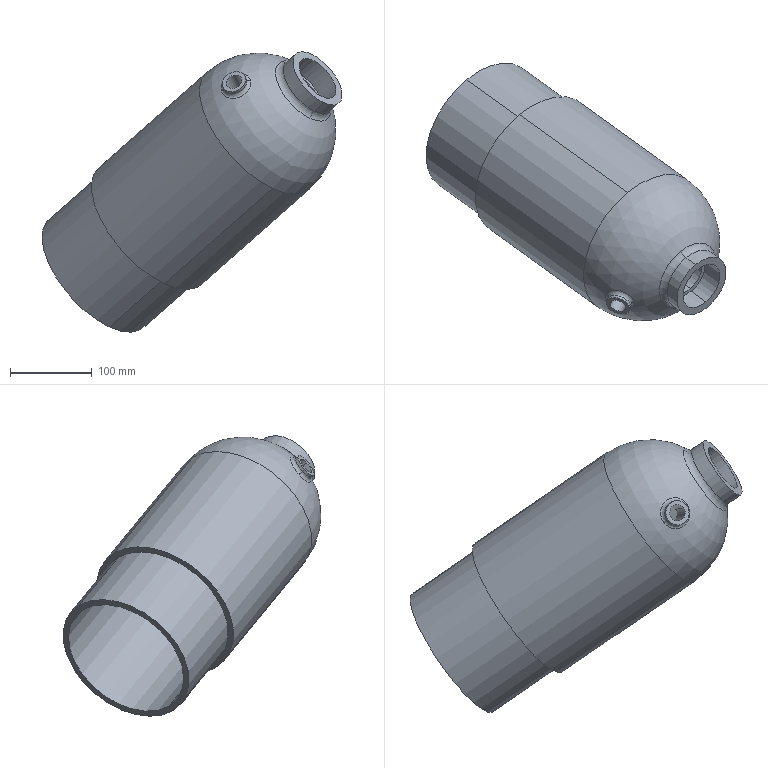Component | SolidWorks | SpringSleeve-1 | 1 solid | 35 faces | box 366.15 x 314.84 x 342.25 mm | volume 2832713 mm3 | cylinder 18 | torus 8 | plane 7 | sphere 2 | commonest cylinder face diameters 30 x4 20 x2 60 x2 175 x2 80 x2 160 x2 190 x2 50 x2 | material 201.0-T7 Insulated Mold Casting (SS)
STEP:
#1=COLOUR_RGB('',0.7922,0.8196,0.9333);
#2=FILL_AREA_STYLE_COLOUR('',#1);
#3=FILL_AREA_STYLE('',(#2));
#4=SURFACE_STYLE_FILL_AREA(#3);
#5=SURFACE_SIDE_STYLE('',(#4));
#6=SURFACE_STYLE_USAGE(.BOTH.,#5);
#7=PRESENTATION_STYLE_ASSIGNMENT((#6));
#8=CARTESIAN_POINT('',(3.904,-75.784,16.909));
#9=VERTEX_POINT('',#8);
#10=CARTESIAN_POINT('',(5.013,-75.909,17.293));
#11=VERTEX_POINT('',#10);
#12=CARTESIAN_POINT('',(4.459,-75.847,17.101));
#13=DIRECTION('',(0.2892,0.7537,-0.5902));
#14=DIRECTION('',(0.9396,-0.1055,0.3256));
#15=AXIS2_PLACEMENT_3D('',#12,#13,#14);
#16=CIRCLE('',#15,0.5906);
#17=EDGE_CURVE('',#9,#11,#16,.T.);
#18=ORIENTED_EDGE('',*,*,#17,.F.);
#19=CARTESIAN_POINT('',(3.615,-75.901,16.939));
#20=VERTEX_POINT('',#19);
#21=CARTESIAN_POINT('',(3.719,-75.764,16.844));
#22=DIRECTION('',(0.1832,-0.6488,-0.7386));
#23=DIRECTION('',(0.,0.7513,-0.6599));
#24=AXIS2_PLACEMENT_3D('',#21,#22,#23);
#25=CIRCLE('',#24,0.1969);
#26=EDGE_CURVE('',#9,#20,#25,.T.);
#27=ORIENTED_EDGE('',*,*,#26,.T.);
#28=CARTESIAN_POINT('',(5.193,-76.078,17.486));
#29=VERTEX_POINT('',#28);
#30=CARTESIAN_POINT('',(4.404,-75.99,17.213));
#31=DIRECTION('',(-0.2892,-0.7537,0.5902));
#32=DIRECTION('',(0.9396,-0.1055,0.3256));
#33=AXIS2_PLACEMENT_3D('',#30,#31,#32);
#34=CIRCLE('',#33,0.8399);
#35=EDGE_CURVE('',#29,#20,#34,.T.);
#36=ORIENTED_EDGE('',*,*,#35,.F.);
#37=CARTESIAN_POINT('',(5.198,-75.93,17.357));
#38=DIRECTION('',(-0.1832,0.6488,0.7386));
#39=DIRECTION('',(0.,-0.7513,0.6599));
#40=AXIS2_PLACEMENT_3D('',#37,#38,#39);
#41=CIRCLE('',#40,0.1969);
#42=EDGE_CURVE('',#11,#29,#41,.T.);
#43=ORIENTED_EDGE('',*,*,#42,.F.);
#44=EDGE_LOOP('',(#18,#27,#36,#43));
#45=FACE_OUTER_BOUND('',#44,.T.);
#46=CARTESIAN_POINT('',(4.459,-75.847,17.101));
#47=DIRECTION('',(0.2892,0.7537,-0.5902));
#48=DIRECTION('',(0.9396,-0.1055,0.3256));
#49=AXIS2_PLACEMENT_3D('',#46,#47,#48);
#50=TOROIDAL_SURFACE('',#49,0.7874,0.1969);
#51=ADVANCED_FACE('',(#45),#50,.F.);
#52=CARTESIAN_POINT('',(3.519,-76.385,17.341));
#53=VERTEX_POINT('',#52);
#54=CARTESIAN_POINT('',(4.925,-76.543,17.828));
#55=VERTEX_POINT('',#54);
#56=CARTESIAN_POINT('',(4.222,-76.464,17.584));
#57=DIRECTION('',(0.2892,0.7537,-0.5902));
#58=DIRECTION('',(0.9396,-0.1055,0.3256));
#59=AXIS2_PLACEMENT_3D('',#56,#57,#58);
#60=CIRCLE('',#59,0.748);
#61=EDGE_CURVE('',#53,#55,#60,.T.);
#62=ORIENTED_EDGE('',*,*,#61,.F.);
#63=CARTESIAN_POINT('',(3.611,-76.547,17.506));
#64=VERTEX_POINT('',#63);
#65=CARTESIAN_POINT('',(3.426,-76.526,17.442));
#66=DIRECTION('',(0.1832,-0.6488,-0.7386));
#67=DIRECTION('',(0.,0.7513,-0.6599));
#68=AXIS2_PLACEMENT_3D('',#65,#66,#67);
#69=CIRCLE('',#68,0.1969);
#70=EDGE_CURVE('',#53,#64,#69,.T.);
#71=ORIENTED_EDGE('',*,*,#70,.T.);
#72=CARTESIAN_POINT('',(4.721,-76.671,17.89));
#73=VERTEX_POINT('',#72);
#74=CARTESIAN_POINT('',(4.166,-76.609,17.698));
#75=DIRECTION('',(-0.2892,-0.7537,0.5902));
#76=DIRECTION('',(0.9396,-0.1055,0.3256));
#77=AXIS2_PLACEMENT_3D('',#74,#75,#76);
#78=CIRCLE('',#77,0.5906);
#79=EDGE_CURVE('',#73,#64,#78,.T.);
#80=ORIENTED_EDGE('',*,*,#79,.F.);
#81=CARTESIAN_POINT('',(4.906,-76.692,17.954));
#82=DIRECTION('',(-0.1832,0.6488,0.7386));
#83=DIRECTION('',(0.,-0.7513,0.6599));
#84=AXIS2_PLACEMENT_3D('',#81,#82,#83);
#85=CIRCLE('',#84,0.1969);
#86=EDGE_CURVE('',#55,#73,#85,.T.);
#87=ORIENTED_EDGE('',*,*,#86,.F.);
#88=EDGE_LOOP('',(#62,#71,#80,#87));
#89=FACE_OUTER_BOUND('',#88,.T.);
#90=CARTESIAN_POINT('',(4.166,-76.609,17.698));
#91=DIRECTION('',(0.2892,0.7537,-0.5902));
#92=DIRECTION('',(0.9396,-0.1055,0.3256));
#93=AXIS2_PLACEMENT_3D('',#90,#91,#92);
#94=TOROIDAL_SURFACE('',#93,0.7874,0.1969);
#95=ADVANCED_FACE('',(#89),#94,.F.);
#96=CARTESIAN_POINT('',(4.096,-75.785,16.957));
#97=VERTEX_POINT('',#96);
#98=CARTESIAN_POINT('',(4.836,-75.868,17.214));
#99=VERTEX_POINT('',#98);
#100=CARTESIAN_POINT('',(4.466,-75.827,17.085));
#101=DIRECTION('',(0.2892,0.7537,-0.5902));
#102=DIRECTION('',(0.9396,-0.1055,0.3256));
#103=AXIS2_PLACEMENT_3D('',#100,#101,#102);
#104=CIRCLE('',#103,0.3937);
#105=EDGE_CURVE('',#97,#99,#104,.T.);
#106=ORIENTED_EDGE('',*,*,#105,.T.);
#107=CARTESIAN_POINT('',(4.494,-76.759,17.911));
#108=VERTEX_POINT('',#107);
#109=CARTESIAN_POINT('',(4.836,-75.868,17.214));
#110=DIRECTION('',(-0.2892,-0.7537,0.5902));
#111=VECTOR('',#110,39.37);
#112=LINE('',#109,#111);
#113=EDGE_CURVE('',#99,#108,#112,.T.);
#114=ORIENTED_EDGE('',*,*,#113,.T.);
#115=CARTESIAN_POINT('',(3.755,-76.675,17.654));
#116=VERTEX_POINT('',#115);
#117=CARTESIAN_POINT('',(4.125,-76.717,17.782));
#118=DIRECTION('',(0.2892,0.7537,-0.5902));
#119=DIRECTION('',(0.9396,-0.1055,0.3256));
#120=AXIS2_PLACEMENT_3D('',#117,#118,#119);
#121=CIRCLE('',#120,0.3937);
#122=EDGE_CURVE('',#116,#108,#121,.T.);
#123=ORIENTED_EDGE('',*,*,#122,.F.);
#124=CARTESIAN_POINT('',(4.096,-75.785,16.957));
#125=DIRECTION('',(-0.2892,-0.7537,0.5902));
#126=VECTOR('',#125,39.37);
#127=LINE('',#124,#126);
#128=EDGE_CURVE('',#97,#116,#127,.T.);
#129=ORIENTED_EDGE('',*,*,#128,.F.);
#130=EDGE_LOOP('',(#106,#114,#123,#129));
#131=FACE_OUTER_BOUND('',#130,.T.);
#132=CARTESIAN_POINT('',(4.466,-75.827,17.085));
#133=DIRECTION('',(-0.2892,-0.7537,0.5902));
#134=DIRECTION('',(-0.9396,0.1055,-0.3256));
#135=AXIS2_PLACEMENT_3D('',#132,#133,#134);
#136=CYLINDRICAL_SURFACE('',#135,0.3937);
#137=ADVANCED_FACE('',(#131),#136,.F.);
#138=CARTESIAN_POINT('',(4.459,-75.847,17.101));
#139=DIRECTION('',(0.2892,0.7537,-0.5902));
#140=DIRECTION('',(0.9396,-0.1055,0.3256));
#141=AXIS2_PLACEMENT_3D('',#138,#139,#140);
#142=CIRCLE('',#141,0.5906);
#143=EDGE_CURVE('',#11,#9,#142,.T.);
#144=ORIENTED_EDGE('',*,*,#143,.T.);
#145=CARTESIAN_POINT('',(3.911,-75.765,16.893));
#146=VERTEX_POINT('',#145);
#147=CARTESIAN_POINT('',(3.57,-76.655,17.59));
#148=DIRECTION('',(0.2892,0.7537,-0.5902));
#149=VECTOR('',#148,39.37);
#150=LINE('',#147,#149);
#151=EDGE_CURVE('',#9,#146,#150,.T.);
#152=ORIENTED_EDGE('',*,*,#151,.T.);
#153=CARTESIAN_POINT('',(5.021,-75.889,17.278));
#154=VERTEX_POINT('',#153);
#155=CARTESIAN_POINT('',(4.466,-75.827,17.085));
#156=DIRECTION('',(0.2892,0.7537,-0.5902));
#157=DIRECTION('',(0.9396,-0.1055,0.3256));
#158=AXIS2_PLACEMENT_3D('',#155,#156,#157);
#159=CIRCLE('',#158,0.5906);
#160=EDGE_CURVE('',#154,#146,#159,.T.);
#161=ORIENTED_EDGE('',*,*,#160,.F.);
#162=CARTESIAN_POINT('',(4.679,-76.779,17.975));
#163=DIRECTION('',(0.2892,0.7537,-0.5902));
#164=VECTOR('',#163,39.37);
#165=LINE('',#162,#164);
#166=EDGE_CURVE('',#11,#154,#165,.T.);
#167=ORIENTED_EDGE('',*,*,#166,.F.);
#168=EDGE_LOOP('',(#144,#152,#161,#167));
#169=FACE_OUTER_BOUND('',#168,.T.);
#170=CARTESIAN_POINT('',(4.125,-76.717,17.782));
#171=DIRECTION('',(0.2892,0.7537,-0.5902));
#172=DIRECTION('',(0.9396,-0.1055,0.3256));
#173=AXIS2_PLACEMENT_3D('',#170,#171,#172);
#174=CYLINDRICAL_SURFACE('',#173,0.5906);
#175=ADVANCED_FACE('',(#169),#174,.T.);
#176=CARTESIAN_POINT('',(4.679,-76.779,17.975));
#177=VERTEX_POINT('',#176);
#178=CARTESIAN_POINT('',(3.57,-76.655,17.59));
#179=VERTEX_POINT('',#178);
#180=CARTESIAN_POINT('',(4.125,-76.717,17.782));
#181=DIRECTION('',(0.2892,0.7537,-0.5902));
#182=DIRECTION('',(0.9396,-0.1055,0.3256));
#183=AXIS2_PLACEMENT_3D('',#180,#181,#182);
#184=CIRCLE('',#183,0.5906);
#185=EDGE_CURVE('',#177,#179,#184,.T.);
#186=ORIENTED_EDGE('',*,*,#185,.T.);
#187=CARTESIAN_POINT('',(3.57,-76.655,17.59));
#188=DIRECTION('',(0.2892,0.7537,-0.5902));
#189=VECTOR('',#188,39.37);
#190=LINE('',#187,#189);
#191=EDGE_CURVE('',#179,#64,#190,.T.);
#192=ORIENTED_EDGE('',*,*,#191,.T.);
#193=CARTESIAN_POINT('',(4.166,-76.609,17.698));
#194=DIRECTION('',(-0.2892,-0.7537,0.5902));
#195=DIRECTION('',(0.9396,-0.1055,0.3256));
#196=AXIS2_PLACEMENT_3D('',#193,#194,#195);
#197=CIRCLE('',#196,0.5906);
#198=EDGE_CURVE('',#64,#73,#197,.T.);
#199=ORIENTED_EDGE('',*,*,#198,.T.);
#200=CARTESIAN_POINT('',(4.679,-76.779,17.975));
#201=DIRECTION('',(0.2892,0.7537,-0.5902));
#202=VECTOR('',#201,39.37);
#203=LINE('',#200,#202);
#204=EDGE_CURVE('',#177,#73,#203,.T.);
#205=ORIENTED_EDGE('',*,*,#204,.F.);
#206=EDGE_LOOP('',(#186,#192,#199,#205));
#207=FACE_OUTER_BOUND('',#206,.T.);
#208=CARTESIAN_POINT('',(4.125,-76.717,17.782));
#209=DIRECTION('',(0.2892,0.7537,-0.5902));
#210=DIRECTION('',(0.9396,-0.1055,0.3256));
#211=AXIS2_PLACEMENT_3D('',#208,#209,#210);
#212=CYLINDRICAL_SURFACE('',#211,0.5906);
#213=ADVANCED_FACE('',(#207),#212,.T.);
#214=CARTESIAN_POINT('',(7.639,-76.015,16.439));
#215=VERTEX_POINT('',#214);
#216=CARTESIAN_POINT('',(7.206,-74.483,18.183));
#217=VERTEX_POINT('',#216);
#218=CARTESIAN_POINT('',(7.423,-75.249,17.311));
#219=DIRECTION('',(0.6592,-0.4763,0.5818));
#220=DIRECTION('',(-0.1832,0.6488,0.7386));
#221=AXIS2_PLACEMENT_3D('',#218,#219,#220);
#222=CIRCLE('',#221,1.181);
#223=EDGE_CURVE('',#215,#217,#222,.T.);
#224=ORIENTED_EDGE('',*,*,#223,.F.);
#225=CARTESIAN_POINT('',(8.353,-76.531,17.069));
#226=VERTEX_POINT('',#225);
#227=CARTESIAN_POINT('',(7.639,-76.015,16.439));
#228=DIRECTION('',(0.6592,-0.4763,0.5818));
#229=VECTOR('',#228,39.37);
#230=LINE('',#227,#229);
#231=EDGE_CURVE('',#215,#226,#230,.T.);
#232=ORIENTED_EDGE('',*,*,#231,.T.);
#233=CARTESIAN_POINT('',(7.92,-74.999,18.813));
#234=VERTEX_POINT('',#233);
#235=CARTESIAN_POINT('',(8.136,-75.765,17.941));
#236=DIRECTION('',(0.6592,-0.4763,0.5818));
#237=DIRECTION('',(-0.1832,0.6488,0.7386));
#238=AXIS2_PLACEMENT_3D('',#235,#236,#237);
#239=CIRCLE('',#238,1.181);
#240=EDGE_CURVE('',#226,#234,#239,.T.);
#241=ORIENTED_EDGE('',*,*,#240,.T.);
#242=CARTESIAN_POINT('',(7.206,-74.483,18.183));
#243=DIRECTION('',(0.6592,-0.4763,0.5818));
#244=VECTOR('',#243,39.37);
#245=LINE('',#242,#244);
#246=EDGE_CURVE('',#217,#234,#245,.T.);
#247=ORIENTED_EDGE('',*,*,#246,.F.);
#248=EDGE_LOOP('',(#224,#232,#241,#247));
#249=FACE_OUTER_BOUND('',#248,.T.);
#250=CARTESIAN_POINT('',(7.423,-75.249,17.311));
#251=DIRECTION('',(0.6592,-0.4763,0.5818));
#252=DIRECTION('',(-0.1832,0.6488,0.7386));
#253=AXIS2_PLACEMENT_3D('',#250,#251,#252);
#254=CYLINDRICAL_SURFACE('',#253,1.181);
#255=ADVANCED_FACE('',(#249),#254,.F.);
#256=CARTESIAN_POINT('',(7.123,-74.113,18.65));
#257=VERTEX_POINT('',#256);
#258=CARTESIAN_POINT('',(7.776,-76.424,16.019));
#259=VERTEX_POINT('',#258);
#260=CARTESIAN_POINT('',(7.45,-75.269,17.335));
#261=DIRECTION('',(-0.6592,0.4763,-0.5818));
#262=DIRECTION('',(0.1832,-0.6488,-0.7386));
#263=AXIS2_PLACEMENT_3D('',#260,#261,#262);
#264=CIRCLE('',#263,1.781);
#265=EDGE_CURVE('',#257,#259,#264,.T.);
#266=ORIENTED_EDGE('',*,*,#265,.F.);
#267=CARTESIAN_POINT('',(7.389,-74.412,18.699));
#268=VERTEX_POINT('',#267);
#269=CARTESIAN_POINT('',(7.317,-74.156,18.99));
#270=DIRECTION('',(-0.7293,-0.5935,0.3404));
#271=DIRECTION('',(0.6312,-0.7756,0.));
#272=AXIS2_PLACEMENT_3D('',#269,#270,#271);
#273=CIRCLE('',#272,0.3937);
#274=EDGE_CURVE('',#257,#268,#273,.T.);
#275=ORIENTED_EDGE('',*,*,#274,.T.);
#276=CARTESIAN_POINT('',(7.966,-76.455,16.373));
#277=VERTEX_POINT('',#276);
#278=CARTESIAN_POINT('',(7.678,-75.433,17.536));
#279=DIRECTION('',(0.6592,-0.4763,0.5818));
#280=DIRECTION('',(0.1832,-0.6488,-0.7386));
#281=AXIS2_PLACEMENT_3D('',#278,#279,#280);
#282=CIRCLE('',#281,1.575);
#283=EDGE_CURVE('',#277,#268,#282,.T.);
#284=ORIENTED_EDGE('',*,*,#283,.F.);
#285=CARTESIAN_POINT('',(8.038,-76.71,16.082));
#286=DIRECTION('',(0.7293,0.5935,-0.3404));
#287=DIRECTION('',(-0.6312,0.7756,0.));
#288=AXIS2_PLACEMENT_3D('',#285,#286,#287);
#289=CIRCLE('',#288,0.3937);
#290=EDGE_CURVE('',#259,#277,#289,.T.);
#291=ORIENTED_EDGE('',*,*,#290,.F.);
#292=EDGE_LOOP('',(#266,#275,#284,#291));
#293=FACE_OUTER_BOUND('',#292,.T.);
#294=CARTESIAN_POINT('',(7.678,-75.433,17.536));
#295=DIRECTION('',(-0.6592,0.4763,-0.5818));
#296=DIRECTION('',(0.1832,-0.6488,-0.7386));
#297=AXIS2_PLACEMENT_3D('',#294,#295,#296);
#298=TOROIDAL_SURFACE('',#297,1.969,0.3937);
#299=ADVANCED_FACE('',(#293),#298,.F.);
#300=CARTESIAN_POINT('',(6.55,-73.805,17.959));
#301=VERTEX_POINT('',#300);
#302=CARTESIAN_POINT('',(7.127,-75.849,15.632));
#303=VERTEX_POINT('',#302);
#304=CARTESIAN_POINT('',(6.839,-74.827,16.796));
#305=DIRECTION('',(-0.6592,0.4763,-0.5818));
#306=DIRECTION('',(0.1832,-0.6488,-0.7386));
#307=AXIS2_PLACEMENT_3D('',#304,#305,#306);
#308=CIRCLE('',#307,1.575);
#309=EDGE_CURVE('',#301,#303,#308,.T.);
#310=ORIENTED_EDGE('',*,*,#309,.F.);
#311=CARTESIAN_POINT('',(6.452,-73.468,18.336));
#312=VERTEX_POINT('',#311);
#313=CARTESIAN_POINT('',(6.306,-73.497,17.972));
#314=DIRECTION('',(-0.7293,-0.5935,0.3404));
#315=DIRECTION('',(0.6312,-0.7756,0.));
#316=AXIS2_PLACEMENT_3D('',#313,#314,#315);
#317=CIRCLE('',#316,0.3937);
#318=EDGE_CURVE('',#301,#312,#317,.T.);
#319=ORIENTED_EDGE('',*,*,#318,.T.);
#320=CARTESIAN_POINT('',(7.218,-76.18,15.248));
#321=VERTEX_POINT('',#320);
#322=CARTESIAN_POINT('',(6.835,-74.824,16.792));
#323=DIRECTION('',(0.6592,-0.4763,0.5818));
#324=DIRECTION('',(0.1832,-0.6488,-0.7386));
#325=AXIS2_PLACEMENT_3D('',#322,#323,#324);
#326=CIRCLE('',#325,2.09);
#327=EDGE_CURVE('',#321,#312,#326,.T.);
#328=ORIENTED_EDGE('',*,*,#327,.F.);
#329=CARTESIAN_POINT('',(6.976,-75.87,15.27));
#330=DIRECTION('',(0.7293,0.5935,-0.3404));
#331=DIRECTION('',(-0.6312,0.7756,0.));
#332=AXIS2_PLACEMENT_3D('',#329,#330,#331);
#333=CIRCLE('',#332,0.3937);
#334=EDGE_CURVE('',#303,#321,#333,.T.);
#335=ORIENTED_EDGE('',*,*,#334,.F.);
#336=EDGE_LOOP('',(#310,#319,#328,#335));
#337=FACE_OUTER_BOUND('',#336,.T.);
#338=CARTESIAN_POINT('',(6.641,-74.684,16.621));
#339=DIRECTION('',(-0.6592,0.4763,-0.5818));
#340=DIRECTION('',(0.1832,-0.6488,-0.7386));
#341=AXIS2_PLACEMENT_3D('',#338,#339,#340);
#342=TOROIDAL_SURFACE('',#341,1.829,0.3937);
#343=ADVANCED_FACE('',(#337),#342,.F.);
#344=CARTESIAN_POINT('',(-1.874,-70.311,6.005));
#345=VERTEX_POINT('',#344);
#346=CARTESIAN_POINT('',(-3.135,-65.841,11.094));
#347=VERTEX_POINT('',#346);
#348=CARTESIAN_POINT('',(-2.505,-68.076,8.549));
#349=DIRECTION('',(-0.6592,0.4763,-0.5818));
#350=DIRECTION('',(0.1832,-0.6488,-0.7386));
#351=AXIS2_PLACEMENT_3D('',#348,#349,#350);
#352=CIRCLE('',#351,3.445);
#353=EDGE_CURVE('',#345,#347,#352,.T.);
#354=ORIENTED_EDGE('',*,*,#353,.F.);
#355=CARTESIAN_POINT('',(0.7217,-72.186,8.295));
#356=VERTEX_POINT('',#355);
#357=CARTESIAN_POINT('',(-1.874,-70.311,6.005));
#358=DIRECTION('',(0.6592,-0.4763,0.5818));
#359=VECTOR('',#358,39.37);
#360=LINE('',#357,#359);
#361=EDGE_CURVE('',#345,#356,#360,.T.);
#362=ORIENTED_EDGE('',*,*,#361,.T.);
#363=CARTESIAN_POINT('',(-0.5401,-67.716,13.384));
#364=VERTEX_POINT('',#363);
#365=CARTESIAN_POINT('',(0.09081,-69.951,10.84));
#366=DIRECTION('',(-0.6592,0.4763,-0.5818));
#367=DIRECTION('',(0.1832,-0.6488,-0.7386));
#368=AXIS2_PLACEMENT_3D('',#365,#366,#367);
#369=CIRCLE('',#368,3.445);
#370=EDGE_CURVE('',#356,#364,#369,.T.);
#371=ORIENTED_EDGE('',*,*,#370,.T.);
#372=CARTESIAN_POINT('',(-3.135,-65.841,11.094));
#373=DIRECTION('',(0.6592,-0.4763,0.5818));
#374=VECTOR('',#373,39.37);
#375=LINE('',#372,#374);
#376=EDGE_CURVE('',#347,#364,#375,.T.);
#377=ORIENTED_EDGE('',*,*,#376,.F.);
#378=EDGE_LOOP('',(#354,#362,#371,#377));
#379=FACE_OUTER_BOUND('',#378,.T.);
#380=CARTESIAN_POINT('',(-2.505,-68.076,8.549));
#381=DIRECTION('',(0.6592,-0.4763,0.5818));
#382=DIRECTION('',(-0.1832,0.6488,0.7386));
#383=AXIS2_PLACEMENT_3D('',#380,#381,#382);
#384=CYLINDRICAL_SURFACE('',#383,3.445);
#385=ADVANCED_FACE('',(#379),#384,.T.);
#386=CARTESIAN_POINT('',(7.678,-75.433,17.536));
#387=DIRECTION('',(0.6592,-0.4763,0.5818));
#388=DIRECTION('',(0.1832,-0.6488,-0.7386));
#389=AXIS2_PLACEMENT_3D('',#386,#387,#388);
#390=CIRCLE('',#389,1.575);
#391=EDGE_CURVE('',#268,#277,#390,.T.);
#392=ORIENTED_EDGE('',*,*,#391,.T.);
#393=CARTESIAN_POINT('',(8.425,-76.786,16.778));
#394=VERTEX_POINT('',#393);
#395=CARTESIAN_POINT('',(7.127,-75.849,15.632));
#396=DIRECTION('',(0.6592,-0.4763,0.5818));
#397=VECTOR('',#396,39.37);
#398=LINE('',#395,#397);
#399=EDGE_CURVE('',#277,#394,#398,.T.);
#400=ORIENTED_EDGE('',*,*,#399,.T.);
#401=CARTESIAN_POINT('',(7.848,-74.743,19.104));
#402=VERTEX_POINT('',#401);
#403=CARTESIAN_POINT('',(8.136,-75.765,17.941));
#404=DIRECTION('',(-0.6592,0.4763,-0.5818));
#405=DIRECTION('',(0.1832,-0.6488,-0.7386));
#406=AXIS2_PLACEMENT_3D('',#403,#404,#405);
#407=CIRCLE('',#406,1.575);
#408=EDGE_CURVE('',#394,#402,#407,.T.);
#409=ORIENTED_EDGE('',*,*,#408,.T.);
#410=CARTESIAN_POINT('',(6.55,-73.805,17.959));
#411=DIRECTION('',(0.6592,-0.4763,0.5818));
#412=VECTOR('',#411,39.37);
#413=LINE('',#410,#412);
#414=EDGE_CURVE('',#268,#402,#413,.T.);
#415=ORIENTED_EDGE('',*,*,#414,.F.);
#416=EDGE_LOOP('',(#392,#400,#409,#415));
#417=FACE_OUTER_BOUND('',#416,.T.);
#418=CARTESIAN_POINT('',(6.839,-74.827,16.796));
#419=DIRECTION('',(0.6592,-0.4763,0.5818));
#420=DIRECTION('',(-0.1832,0.6488,0.7386));
#421=AXIS2_PLACEMENT_3D('',#418,#419,#420);
#422=CYLINDRICAL_SURFACE('',#421,1.575);
#423=ADVANCED_FACE('',(#417),#422,.T.);
#424=CARTESIAN_POINT('',(-3.081,-66.033,10.875));
#425=VERTEX_POINT('',#424);
#426=CARTESIAN_POINT('',(-1.928,-70.119,6.223));
#427=VERTEX_POINT('',#426);
#428=CARTESIAN_POINT('',(-2.505,-68.076,8.549));
#429=DIRECTION('',(-0.6592,0.4763,-0.5818));
#430=DIRECTION('',(0.1832,-0.6488,-0.7386));
#431=AXIS2_PLACEMENT_3D('',#428,#429,#430);
#432=CIRCLE('',#431,3.15);
#433=EDGE_CURVE('',#425,#427,#432,.T.);
#434=ORIENTED_EDGE('',*,*,#433,.T.);
#435=CARTESIAN_POINT('',(5.858,-75.745,13.095));
#436=VERTEX_POINT('',#435);
#437=CARTESIAN_POINT('',(-1.928,-70.119,6.223));
#438=DIRECTION('',(0.6592,-0.4763,0.5818));
#439=VECTOR('',#438,39.37);
#440=LINE('',#437,#439);
#441=EDGE_CURVE('',#427,#436,#440,.T.);
#442=ORIENTED_EDGE('',*,*,#441,.T.);
#443=CARTESIAN_POINT('',(4.705,-71.659,17.748));
#444=VERTEX_POINT('',#443);
#445=CARTESIAN_POINT('',(5.282,-73.702,15.421));
#446=DIRECTION('',(-0.6592,0.4763,-0.5818));
#447=DIRECTION('',(0.1832,-0.6488,-0.7386));
#448=AXIS2_PLACEMENT_3D('',#445,#446,#447);
#449=CIRCLE('',#448,3.15);
#450=EDGE_CURVE('',#444,#436,#449,.T.);
#451=ORIENTED_EDGE('',*,*,#450,.F.);
#452=CARTESIAN_POINT('',(-3.081,-66.033,10.875));
#453=DIRECTION('',(0.6592,-0.4763,0.5818));
#454=VECTOR('',#453,39.37);
#455=LINE('',#452,#454);
#456=EDGE_CURVE('',#425,#444,#455,.T.);
#457=ORIENTED_EDGE('',*,*,#456,.F.);
#458=EDGE_LOOP('',(#434,#442,#451,#457));
#459=FACE_OUTER_BOUND('',#458,.T.);
#460=CARTESIAN_POINT('',(-2.505,-68.076,8.549));
#461=DIRECTION('',(0.6592,-0.4763,0.5818));
#462=DIRECTION('',(-0.1832,0.6488,0.7386));
#463=AXIS2_PLACEMENT_3D('',#460,#461,#462);
#464=CYLINDRICAL_SURFACE('',#463,3.15);
#465=ADVANCED_FACE('',(#459),#464,.F.);
#466=CARTESIAN_POINT('',(0.7758,-72.378,8.077));
#467=VERTEX_POINT('',#466);
#468=CARTESIAN_POINT('',(-0.5942,-67.525,13.602));
#469=VERTEX_POINT('',#468);
#470=CARTESIAN_POINT('',(0.09081,-69.951,10.84));
#471=DIRECTION('',(-0.6592,0.4763,-0.5818));
#472=DIRECTION('',(0.1832,-0.6488,-0.7386));
#473=AXIS2_PLACEMENT_3D('',#470,#471,#472);
#474=CIRCLE('',#473,3.74);
#475=EDGE_CURVE('',#467,#469,#474,.T.);
#476=ORIENTED_EDGE('',*,*,#475,.F.);
#477=CARTESIAN_POINT('',(5.967,-76.128,12.659));
#478=VERTEX_POINT('',#477);
#479=CARTESIAN_POINT('',(-1.82,-70.502,5.786));
#480=DIRECTION('',(0.6592,-0.4763,0.5818));
#481=VECTOR('',#480,39.37);
#482=LINE('',#479,#481);
#483=EDGE_CURVE('',#467,#478,#482,.T.);
#484=ORIENTED_EDGE('',*,*,#483,.T.);
#485=CARTESIAN_POINT('',(4.597,-71.275,18.184));
#486=VERTEX_POINT('',#485);
#487=CARTESIAN_POINT('',(5.282,-73.702,15.421));
#488=DIRECTION('',(-0.6592,0.4763,-0.5818));
#489=DIRECTION('',(0.7293,0.5935,-0.3404));
#490=AXIS2_PLACEMENT_3D('',#487,#488,#489);
#491=CIRCLE('',#490,3.74);
#492=EDGE_CURVE('',#478,#486,#491,.T.);
#493=ORIENTED_EDGE('',*,*,#492,.T.);
#494=CARTESIAN_POINT('',(-3.19,-65.649,11.312));
#495=DIRECTION('',(0.6592,-0.4763,0.5818));
#496=VECTOR('',#495,39.37);
#497=LINE('',#494,#496);
#498=EDGE_CURVE('',#469,#486,#497,.T.);
#499=ORIENTED_EDGE('',*,*,#498,.F.);
#500=EDGE_LOOP('',(#476,#484,#493,#499));
#501=FACE_OUTER_BOUND('',#500,.T.);
#502=CARTESIAN_POINT('',(-2.505,-68.076,8.549));
#503=DIRECTION('',(0.6592,-0.4763,0.5818));
#504=DIRECTION('',(-0.1832,0.6488,0.7386));
#505=AXIS2_PLACEMENT_3D('',#502,#503,#504);
#506=CYLINDRICAL_SURFACE('',#505,3.74);
#507=ADVANCED_FACE('',(#501),#506,.T.);
#508=CARTESIAN_POINT('',(6.658,-74.189,17.523));
#509=VERTEX_POINT('',#508);
#510=CARTESIAN_POINT('',(7.019,-75.466,16.069));
#511=VERTEX_POINT('',#510);
#512=CARTESIAN_POINT('',(6.839,-74.827,16.796));
#513=DIRECTION('',(-0.6592,0.4763,-0.5818));
#514=DIRECTION('',(0.1832,-0.6488,-0.7386));
#515=AXIS2_PLACEMENT_3D('',#512,#513,#514);
#516=CIRCLE('',#515,0.9843);
#517=EDGE_CURVE('',#509,#511,#516,.T.);
#518=ORIENTED_EDGE('',*,*,#517,.T.);
#519=CARTESIAN_POINT('',(7.603,-75.888,16.584));
#520=VERTEX_POINT('',#519);
#521=CARTESIAN_POINT('',(6.63,-75.184,15.725));
#522=DIRECTION('',(0.6592,-0.4763,0.5818));
#523=VECTOR('',#522,39.37);
#524=LINE('',#521,#523);
#525=EDGE_CURVE('',#511,#520,#524,.T.);
#526=ORIENTED_EDGE('',*,*,#525,.T.);
#527=CARTESIAN_POINT('',(7.242,-74.611,18.038));
#528=VERTEX_POINT('',#527);
#529=CARTESIAN_POINT('',(7.423,-75.249,17.311));
#530=DIRECTION('',(-0.6592,0.4763,-0.5818));
#531=DIRECTION('',(-0.1832,0.6488,0.7386));
#532=AXIS2_PLACEMENT_3D('',#529,#530,#531);
#533=CIRCLE('',#532,0.9843);
#534=EDGE_CURVE('',#528,#520,#533,.T.);
#535=ORIENTED_EDGE('',*,*,#534,.F.);
#536=CARTESIAN_POINT('',(6.269,-73.907,17.179));
#537=DIRECTION('',(0.6592,-0.4763,0.5818));
#538=VECTOR('',#537,39.37);
#539=LINE('',#536,#538);
#540=EDGE_CURVE('',#509,#528,#539,.T.);
#541=ORIENTED_EDGE('',*,*,#540,.F.);
#542=EDGE_LOOP('',(#518,#526,#535,#541));
#543=FACE_OUTER_BOUND('',#542,.T.);
#544=CARTESIAN_POINT('',(6.449,-74.546,16.452));
#545=DIRECTION('',(0.6592,-0.4763,0.5818));
#546=DIRECTION('',(-0.1832,0.6488,0.7386));
#547=AXIS2_PLACEMENT_3D('',#544,#545,#546);
#548=CYLINDRICAL_SURFACE('',#547,0.9843);
#549=ADVANCED_FACE('',(#543),#548,.F.);
#550=ORIENTED_EDGE('',*,*,#525,.F.);
#551=CARTESIAN_POINT('',(6.839,-74.827,16.796));
#552=DIRECTION('',(-0.6592,0.4763,-0.5818));
#553=DIRECTION('',(0.1832,-0.6488,-0.7386));
#554=AXIS2_PLACEMENT_3D('',#551,#552,#553);
#555=CIRCLE('',#554,0.9843);
#556=EDGE_CURVE('',#511,#509,#555,.T.);
#557=ORIENTED_EDGE('',*,*,#556,.T.);
#558=ORIENTED_EDGE('',*,*,#540,.T.);
#559=CARTESIAN_POINT('',(7.423,-75.249,17.311));
#560=DIRECTION('',(-0.6592,0.4763,-0.5818));
#561=DIRECTION('',(-0.1832,0.6488,0.7386));
#562=AXIS2_PLACEMENT_3D('',#559,#560,#561);
#563=CIRCLE('',#562,0.9843);
#564=EDGE_CURVE('',#520,#528,#563,.T.);
#565=ORIENTED_EDGE('',*,*,#564,.F.);
#566=EDGE_LOOP('',(#550,#557,#558,#565));
#567=FACE_OUTER_BOUND('',#566,.T.);
#568=CARTESIAN_POINT('',(6.449,-74.546,16.452));
#569=DIRECTION('',(0.6592,-0.4763,0.5818));
#570=DIRECTION('',(-0.1832,0.6488,0.7386));
#571=AXIS2_PLACEMENT_3D('',#568,#569,#570);
#572=CYLINDRICAL_SURFACE('',#571,0.9843);
#573=ADVANCED_FACE('',(#567),#572,.F.);
#574=ORIENTED_EDGE('',*,*,#433,.F.);
#575=CARTESIAN_POINT('',(-2.505,-68.076,8.549));
#576=DIRECTION('',(-0.6592,0.4763,-0.5818));
#577=DIRECTION('',(0.1832,-0.6488,-0.7386));
#578=AXIS2_PLACEMENT_3D('',#575,#576,#577);
#579=CIRCLE('',#578,3.15);
#580=EDGE_CURVE('',#427,#425,#579,.T.);
#581=ORIENTED_EDGE('',*,*,#580,.F.);
#582=EDGE_LOOP('',(#574,#581));
#583=FACE_BOUND('',#582,.T.);
#584=CARTESIAN_POINT('',(-2.505,-68.076,8.549));
#585=DIRECTION('',(-0.6592,0.4763,-0.5818));
#586=DIRECTION('',(0.1832,-0.6488,-0.7386));
#587=AXIS2_PLACEMENT_3D('',#584,#585,#586);
#588=CIRCLE('',#587,3.445);
#589=EDGE_CURVE('',#347,#345,#588,.T.);
#590=ORIENTED_EDGE('',*,*,#589,.T.);
#591=ORIENTED_EDGE('',*,*,#353,.T.);
#592=EDGE_LOOP('',(#590,#591));
#593=FACE_OUTER_BOUND('',#592,.T.);
#594=CARTESIAN_POINT('',(-2.505,-68.076,8.549));
#595=DIRECTION('',(-0.6592,0.4763,-0.5818));
#596=DIRECTION('',(0.1832,-0.6488,-0.7386));
#597=AXIS2_PLACEMENT_3D('',#594,#595,#596);
#598=PLANE('',#597);
#599=ADVANCED_FACE('',(#583,#593),#598,.T.);
#600=ORIENTED_EDGE('',*,*,#483,.F.);
#601=CARTESIAN_POINT('',(0.09081,-69.951,10.84));
#602=DIRECTION('',(-0.6592,0.4763,-0.5818));
#603=DIRECTION('',(0.1832,-0.6488,-0.7386));
#604=AXIS2_PLACEMENT_3D('',#601,#602,#603);
#605=CIRCLE('',#604,3.74);
#606=EDGE_CURVE('',#469,#467,#605,.T.);
#607=ORIENTED_EDGE('',*,*,#606,.F.);
#608=ORIENTED_EDGE('',*,*,#498,.T.);
#609=CARTESIAN_POINT('',(5.282,-73.702,15.421));
#610=DIRECTION('',(-0.6592,0.4763,-0.5818));
#611=DIRECTION('',(0.7293,0.5935,-0.3404));
#612=AXIS2_PLACEMENT_3D('',#609,#610,#611);
#613=CIRCLE('',#612,3.74);
#614=EDGE_CURVE('',#486,#478,#613,.T.);
#615=ORIENTED_EDGE('',*,*,#614,.T.);
#616=EDGE_LOOP('',(#600,#607,#608,#615));
#617=FACE_OUTER_BOUND('',#616,.T.);
#618=CARTESIAN_POINT('',(-2.505,-68.076,8.549));
#619=DIRECTION('',(0.6592,-0.4763,0.5818));
#620=DIRECTION('',(-0.1832,0.6488,0.7386));
#621=AXIS2_PLACEMENT_3D('',#618,#619,#620);
#622=CYLINDRICAL_SURFACE('',#621,3.74);
#623=ADVANCED_FACE('',(#617),#622,.T.);
#624=ORIENTED_EDGE('',*,*,#35,.T.);
#625=CARTESIAN_POINT('',(4.404,-75.99,17.213));
#626=DIRECTION('',(-0.2892,-0.7537,0.5902));
#627=DIRECTION('',(0.9396,-0.1055,0.3256));
#628=AXIS2_PLACEMENT_3D('',#625,#626,#627);
#629=CIRCLE('',#628,0.8399);
#630=EDGE_CURVE('',#20,#29,#629,.T.);
#631=ORIENTED_EDGE('',*,*,#630,.T.);
#632=EDGE_LOOP('',(#624,#631));
#633=FACE_BOUND('',#632,.T.);
#634=ORIENTED_EDGE('',*,*,#327,.T.);
#635=CARTESIAN_POINT('',(6.835,-74.824,16.792));
#636=DIRECTION('',(0.6592,-0.4763,0.5818));
#637=DIRECTION('',(0.1832,-0.6488,-0.7386));
#638=AXIS2_PLACEMENT_3D('',#635,#636,#637);
#639=CIRCLE('',#638,2.09);
#640=EDGE_CURVE('',#312,#321,#639,.T.);
#641=ORIENTED_EDGE('',*,*,#640,.T.);
#642=EDGE_LOOP('',(#634,#641));
#643=FACE_BOUND('',#642,.T.);
#644=ORIENTED_EDGE('',*,*,#450,.T.);
#645=CARTESIAN_POINT('',(5.282,-73.702,15.421));
#646=DIRECTION('',(-0.6592,0.4763,-0.5818));
#647=DIRECTION('',(0.1832,-0.6488,-0.7386));
#648=AXIS2_PLACEMENT_3D('',#645,#646,#647);
#649=CIRCLE('',#648,3.15);
#650=EDGE_CURVE('',#436,#444,#649,.T.);
#651=ORIENTED_EDGE('',*,*,#650,.T.);
#652=EDGE_LOOP('',(#644,#651));
#653=FACE_OUTER_BOUND('',#652,.T.);
#654=CARTESIAN_POINT('',(5.282,-73.702,15.421));
#655=DIRECTION('',(-0.6592,0.4763,-0.5818));
#656=DIRECTION('',(0.1832,-0.6488,-0.7386));
#657=AXIS2_PLACEMENT_3D('',#654,#655,#656);
#658=SPHERICAL_SURFACE('',#657,3.15);
#659=ADVANCED_FACE('',(#633,#643,#653),#658,.F.);
#660=CARTESIAN_POINT('',(4.222,-76.464,17.584));
#661=DIRECTION('',(0.2892,0.7537,-0.5902));
#662=DIRECTION('',(0.9396,-0.1055,0.3256));
#663=AXIS2_PLACEMENT_3D('',#660,#661,#662);
#664=CIRCLE('',#663,0.748);
#665=EDGE_CURVE('',#55,#53,#664,.T.);
#666=ORIENTED_EDGE('',*,*,#665,.T.);
#667=ORIENTED_EDGE('',*,*,#61,.T.);
#668=EDGE_LOOP('',(#666,#667));
#669=FACE_BOUND('',#668,.T.);
#670=CARTESIAN_POINT('',(7.45,-75.269,17.335));
#671=DIRECTION('',(-0.6592,0.4763,-0.5818));
#672=DIRECTION('',(0.1832,-0.6488,-0.7386));
#673=AXIS2_PLACEMENT_3D('',#670,#671,#672);
#674=CIRCLE('',#673,1.781);
#675=EDGE_CURVE('',#259,#257,#674,.T.);
#676=ORIENTED_EDGE('',*,*,#675,.T.);
#677=ORIENTED_EDGE('',*,*,#265,.T.);
#678=EDGE_LOOP('',(#676,#677));
#679=FACE_BOUND('',#678,.T.);
#680=ORIENTED_EDGE('',*,*,#614,.F.);
#681=ORIENTED_EDGE('',*,*,#492,.F.);
#682=EDGE_LOOP('',(#680,#681));
#683=FACE_OUTER_BOUND('',#682,.T.);
#684=CARTESIAN_POINT('',(5.282,-73.702,15.421));
#685=DIRECTION('',(-0.6592,0.4763,-0.5818));
#686=DIRECTION('',(0.1832,-0.6488,-0.7386));
#687=AXIS2_PLACEMENT_3D('',#684,#685,#686);
#688=SPHERICAL_SURFACE('',#687,3.74);
#689=ADVANCED_FACE('',(#669,#679,#683),#688,.T.);
#690=ORIENTED_EDGE('',*,*,#441,.F.);
#691=ORIENTED_EDGE('',*,*,#580,.T.);
#692=ORIENTED_EDGE('',*,*,#456,.T.);
#693=ORIENTED_EDGE('',*,*,#650,.F.);
#694=EDGE_LOOP('',(#690,#691,#692,#693));
#695=FACE_OUTER_BOUND('',#694,.T.);
#696=CARTESIAN_POINT('',(-2.505,-68.076,8.549));
#697=DIRECTION('',(0.6592,-0.4763,0.5818));
#698=DIRECTION('',(-0.1832,0.6488,0.7386));
#699=AXIS2_PLACEMENT_3D('',#696,#697,#698);
#700=CYLINDRICAL_SURFACE('',#699,3.15);
#701=ADVANCED_FACE('',(#695),#700,.F.);
#702=ORIENTED_EDGE('',*,*,#399,.F.);
#703=ORIENTED_EDGE('',*,*,#283,.T.);
#704=ORIENTED_EDGE('',*,*,#414,.T.);
#705=CARTESIAN_POINT('',(8.136,-75.765,17.941));
#706=DIRECTION('',(-0.6592,0.4763,-0.5818));
#707=DIRECTION('',(0.1832,-0.6488,-0.7386));
#708=AXIS2_PLACEMENT_3D('',#705,#706,#707);
#709=CIRCLE('',#708,1.575);
#710=EDGE_CURVE('',#402,#394,#709,.T.);
#711=ORIENTED_EDGE('',*,*,#710,.T.);
#712=EDGE_LOOP('',(#702,#703,#704,#711));
#713=FACE_OUTER_BOUND('',#712,.T.);
#714=CARTESIAN_POINT('',(6.839,-74.827,16.796));
#715=DIRECTION('',(0.6592,-0.4763,0.5818));
#716=DIRECTION('',(-0.1832,0.6488,0.7386));
#717=AXIS2_PLACEMENT_3D('',#714,#715,#716);
#718=CYLINDRICAL_SURFACE('',#717,1.575);
#719=ADVANCED_FACE('',(#713),#718,.T.);
#720=CARTESIAN_POINT('',(8.136,-75.765,17.941));
#721=DIRECTION('',(0.6592,-0.4763,0.5818));
#722=DIRECTION('',(-0.1832,0.6488,0.7386));
#723=AXIS2_PLACEMENT_3D('',#720,#721,#722);
#724=CIRCLE('',#723,1.181);
#725=EDGE_CURVE('',#234,#226,#724,.T.);
#726=ORIENTED_EDGE('',*,*,#725,.F.);
#727=ORIENTED_EDGE('',*,*,#240,.F.);
#728=EDGE_LOOP('',(#726,#727));
#729=FACE_BOUND('',#728,.T.);
#730=ORIENTED_EDGE('',*,*,#710,.F.);
#731=ORIENTED_EDGE('',*,*,#408,.F.);
#732=EDGE_LOOP('',(#730,#731));
#733=FACE_OUTER_BOUND('',#732,.T.);
#734=CARTESIAN_POINT('',(8.136,-75.765,17.941));
#735=DIRECTION('',(-0.6592,0.4763,-0.5818));
#736=DIRECTION('',(0.1832,-0.6488,-0.7386));
#737=AXIS2_PLACEMENT_3D('',#734,#735,#736);
#738=PLANE('',#737);
#739=ADVANCED_FACE('',(#729,#733),#738,.F.);
#740=CARTESIAN_POINT('',(6.839,-74.827,16.796));
#741=DIRECTION('',(-0.6592,0.4763,-0.5818));
#742=DIRECTION('',(0.1832,-0.6488,-0.7386));
#743=AXIS2_PLACEMENT_3D('',#740,#741,#742);
#744=CIRCLE('',#743,1.575);
#745=EDGE_CURVE('',#303,#301,#744,.T.);
#746=ORIENTED_EDGE('',*,*,#745,.T.);
#747=ORIENTED_EDGE('',*,*,#309,.T.);
#748=EDGE_LOOP('',(#746,#747));
#749=FACE_OUTER_BOUND('',#748,.T.);
#750=ORIENTED_EDGE('',*,*,#517,.F.);
#751=ORIENTED_EDGE('',*,*,#556,.F.);
#752=EDGE_LOOP('',(#750,#751));
#753=FACE_BOUND('',#752,.T.);
#754=CARTESIAN_POINT('',(6.839,-74.827,16.796));
#755=DIRECTION('',(-0.6592,0.4763,-0.5818));
#756=DIRECTION('',(0.1832,-0.6488,-0.7386));
#757=AXIS2_PLACEMENT_3D('',#754,#755,#756);
#758=PLANE('',#757);
#759=ADVANCED_FACE('',(#749,#753),#758,.T.);
#760=CARTESIAN_POINT('',(0.09081,-69.951,10.84));
#761=DIRECTION('',(-0.6592,0.4763,-0.5818));
#762=DIRECTION('',(0.1832,-0.6488,-0.7386));
#763=AXIS2_PLACEMENT_3D('',#760,#761,#762);
#764=CIRCLE('',#763,3.445);
#765=EDGE_CURVE('',#364,#356,#764,.T.);
#766=ORIENTED_EDGE('',*,*,#765,.F.);
#767=ORIENTED_EDGE('',*,*,#370,.F.);
#768=EDGE_LOOP('',(#766,#767));
#769=FACE_BOUND('',#768,.T.);
#770=ORIENTED_EDGE('',*,*,#606,.T.);
#771=ORIENTED_EDGE('',*,*,#475,.T.);
#772=EDGE_LOOP('',(#770,#771));
#773=FACE_OUTER_BOUND('',#772,.T.);
#774=CARTESIAN_POINT('',(0.09081,-69.951,10.84));
#775=DIRECTION('',(-0.6592,0.4763,-0.5818));
#776=DIRECTION('',(0.1832,-0.6488,-0.7386));
#777=AXIS2_PLACEMENT_3D('',#774,#775,#776);
#778=PLANE('',#777);
#779=ADVANCED_FACE('',(#769,#773),#778,.T.);
#780=ORIENTED_EDGE('',*,*,#361,.F.);
#781=ORIENTED_EDGE('',*,*,#589,.F.);
#782=ORIENTED_EDGE('',*,*,#376,.T.);
#783=ORIENTED_EDGE('',*,*,#765,.T.);
#784=EDGE_LOOP('',(#780,#781,#782,#783));
#785=FACE_OUTER_BOUND('',#784,.T.);
#786=CARTESIAN_POINT('',(-2.505,-68.076,8.549));
#787=DIRECTION('',(0.6592,-0.4763,0.5818));
#788=DIRECTION('',(-0.1832,0.6488,0.7386));
#789=AXIS2_PLACEMENT_3D('',#786,#787,#788);
#790=CYLINDRICAL_SURFACE('',#789,3.445);
#791=ADVANCED_FACE('',(#785),#790,.T.);
#792=ORIENTED_EDGE('',*,*,#318,.F.);
#793=ORIENTED_EDGE('',*,*,#745,.F.);
#794=ORIENTED_EDGE('',*,*,#334,.T.);
#795=ORIENTED_EDGE('',*,*,#640,.F.);
#796=EDGE_LOOP('',(#792,#793,#794,#795));
#797=FACE_OUTER_BOUND('',#796,.T.);
#798=CARTESIAN_POINT('',(6.641,-74.684,16.621));
#799=DIRECTION('',(-0.6592,0.4763,-0.5818));
#800=DIRECTION('',(0.1832,-0.6488,-0.7386));
#801=AXIS2_PLACEMENT_3D('',#798,#799,#800);
#802=TOROIDAL_SURFACE('',#801,1.829,0.3937);
#803=ADVANCED_FACE('',(#797),#802,.F.);
#804=ORIENTED_EDGE('',*,*,#274,.F.);
#805=ORIENTED_EDGE('',*,*,#675,.F.);
#806=ORIENTED_EDGE('',*,*,#290,.T.);
#807=ORIENTED_EDGE('',*,*,#391,.F.);
#808=EDGE_LOOP('',(#804,#805,#806,#807));
#809=FACE_OUTER_BOUND('',#808,.T.);
#810=CARTESIAN_POINT('',(7.678,-75.433,17.536));
#811=DIRECTION('',(-0.6592,0.4763,-0.5818));
#812=DIRECTION('',(0.1832,-0.6488,-0.7386));
#813=AXIS2_PLACEMENT_3D('',#810,#811,#812);
#814=TOROIDAL_SURFACE('',#813,1.969,0.3937);
#815=ADVANCED_FACE('',(#809),#814,.F.);
#816=CARTESIAN_POINT('',(7.423,-75.249,17.311));
#817=DIRECTION('',(0.6592,-0.4763,0.5818));
#818=DIRECTION('',(-0.1832,0.6488,0.7386));
#819=AXIS2_PLACEMENT_3D('',#816,#817,#818);
#820=CIRCLE('',#819,1.181);
#821=EDGE_CURVE('',#217,#215,#820,.T.);
#822=ORIENTED_EDGE('',*,*,#821,.T.);
#823=ORIENTED_EDGE('',*,*,#223,.T.);
#824=EDGE_LOOP('',(#822,#823));
#825=FACE_OUTER_BOUND('',#824,.T.);
#826=ORIENTED_EDGE('',*,*,#534,.T.);
#827=ORIENTED_EDGE('',*,*,#564,.T.);
#828=EDGE_LOOP('',(#826,#827));
#829=FACE_BOUND('',#828,.T.);
#830=CARTESIAN_POINT('',(7.423,-75.249,17.311));
#831=DIRECTION('',(0.6592,-0.4763,0.5818));
#832=DIRECTION('',(-0.1832,0.6488,0.7386));
#833=AXIS2_PLACEMENT_3D('',#830,#831,#832);
#834=PLANE('',#833);
#835=ADVANCED_FACE('',(#825,#829),#834,.T.);
#836=ORIENTED_EDGE('',*,*,#231,.F.);
#837=ORIENTED_EDGE('',*,*,#821,.F.);
#838=ORIENTED_EDGE('',*,*,#246,.T.);
#839=ORIENTED_EDGE('',*,*,#725,.T.);
#840=EDGE_LOOP('',(#836,#837,#838,#839));
#841=FACE_OUTER_BOUND('',#840,.T.);
#842=CARTESIAN_POINT('',(7.423,-75.249,17.311));
#843=DIRECTION('',(0.6592,-0.4763,0.5818));
#844=DIRECTION('',(-0.1832,0.6488,0.7386));
#845=AXIS2_PLACEMENT_3D('',#842,#843,#844);
#846=CYLINDRICAL_SURFACE('',#845,1.181);
#847=ADVANCED_FACE('',(#841),#846,.F.);
#848=ORIENTED_EDGE('',*,*,#122,.T.);
#849=CARTESIAN_POINT('',(4.125,-76.717,17.782));
#850=DIRECTION('',(0.2892,0.7537,-0.5902));
#851=DIRECTION('',(0.9396,-0.1055,0.3256));
#852=AXIS2_PLACEMENT_3D('',#849,#850,#851);
#853=CIRCLE('',#852,0.3937);
#854=EDGE_CURVE('',#108,#116,#853,.T.);
#855=ORIENTED_EDGE('',*,*,#854,.T.);
#856=EDGE_LOOP('',(#848,#855));
#857=FACE_BOUND('',#856,.T.);
#858=ORIENTED_EDGE('',*,*,#185,.F.);
#859=CARTESIAN_POINT('',(4.125,-76.717,17.782));
#860=DIRECTION('',(0.2892,0.7537,-0.5902));
#861=DIRECTION('',(0.9396,-0.1055,0.3256));
#862=AXIS2_PLACEMENT_3D('',#859,#860,#861);
#863=CIRCLE('',#862,0.5906);
#864=EDGE_CURVE('',#179,#177,#863,.T.);
#865=ORIENTED_EDGE('',*,*,#864,.F.);
#866=EDGE_LOOP('',(#858,#865));
#867=FACE_OUTER_BOUND('',#866,.T.);
#868=CARTESIAN_POINT('',(4.125,-76.717,17.782));
#869=DIRECTION('',(0.2892,0.7537,-0.5902));
#870=DIRECTION('',(0.9396,-0.1055,0.3256));
#871=AXIS2_PLACEMENT_3D('',#868,#869,#870);
#872=PLANE('',#871);
#873=ADVANCED_FACE('',(#857,#867),#872,.F.);
#874=ORIENTED_EDGE('',*,*,#191,.F.);
#875=ORIENTED_EDGE('',*,*,#864,.T.);
#876=ORIENTED_EDGE('',*,*,#204,.T.);
#877=ORIENTED_EDGE('',*,*,#79,.T.);
#878=EDGE_LOOP('',(#874,#875,#876,#877));
#879=FACE_OUTER_BOUND('',#878,.T.);
#880=CARTESIAN_POINT('',(4.125,-76.717,17.782));
#881=DIRECTION('',(0.2892,0.7537,-0.5902));
#882=DIRECTION('',(0.9396,-0.1055,0.3256));
#883=AXIS2_PLACEMENT_3D('',#880,#881,#882);
#884=CYLINDRICAL_SURFACE('',#883,0.5906);
#885=ADVANCED_FACE('',(#879),#884,.T.);
#886=ORIENTED_EDGE('',*,*,#151,.F.);
#887=ORIENTED_EDGE('',*,*,#17,.T.);
#888=ORIENTED_EDGE('',*,*,#166,.T.);
#889=CARTESIAN_POINT('',(4.466,-75.827,17.085));
#890=DIRECTION('',(0.2892,0.7537,-0.5902));
#891=DIRECTION('',(0.9396,-0.1055,0.3256));
#892=AXIS2_PLACEMENT_3D('',#889,#890,#891);
#893=CIRCLE('',#892,0.5906);
#894=EDGE_CURVE('',#146,#154,#893,.T.);
#895=ORIENTED_EDGE('',*,*,#894,.F.);
#896=EDGE_LOOP('',(#886,#887,#888,#895));
#897=FACE_OUTER_BOUND('',#896,.T.);
#898=CARTESIAN_POINT('',(4.125,-76.717,17.782));
#899=DIRECTION('',(0.2892,0.7537,-0.5902));
#900=DIRECTION('',(0.9396,-0.1055,0.3256));
#901=AXIS2_PLACEMENT_3D('',#898,#899,#900);
#902=CYLINDRICAL_SURFACE('',#901,0.5906);
#903=ADVANCED_FACE('',(#897),#902,.T.);
#904=ORIENTED_EDGE('',*,*,#105,.F.);
#905=CARTESIAN_POINT('',(4.466,-75.827,17.085));
#906=DIRECTION('',(0.2892,0.7537,-0.5902));
#907=DIRECTION('',(0.9396,-0.1055,0.3256));
#908=AXIS2_PLACEMENT_3D('',#905,#906,#907);
#909=CIRCLE('',#908,0.3937);
#910=EDGE_CURVE('',#99,#97,#909,.T.);
#911=ORIENTED_EDGE('',*,*,#910,.F.);
#912=EDGE_LOOP('',(#904,#911));
#913=FACE_BOUND('',#912,.T.);
#914=ORIENTED_EDGE('',*,*,#160,.T.);
#915=ORIENTED_EDGE('',*,*,#894,.T.);
#916=EDGE_LOOP('',(#914,#915));
#917=FACE_OUTER_BOUND('',#916,.T.);
#918=CARTESIAN_POINT('',(4.466,-75.827,17.085));
#919=DIRECTION('',(0.2892,0.7537,-0.5902));
#920=DIRECTION('',(0.9396,-0.1055,0.3256));
#921=AXIS2_PLACEMENT_3D('',#918,#919,#920);
#922=PLANE('',#921);
#923=ADVANCED_FACE('',(#913,#917),#922,.T.);
#924=ORIENTED_EDGE('',*,*,#113,.F.);
#925=ORIENTED_EDGE('',*,*,#910,.T.);
#926=ORIENTED_EDGE('',*,*,#128,.T.);
#927=ORIENTED_EDGE('',*,*,#854,.F.);
#928=EDGE_LOOP('',(#924,#925,#926,#927));
#929=FACE_OUTER_BOUND('',#928,.T.);
#930=CARTESIAN_POINT('',(4.466,-75.827,17.085));
#931=DIRECTION('',(-0.2892,-0.7537,0.5902));
#932=DIRECTION('',(-0.9396,0.1055,-0.3256));
#933=AXIS2_PLACEMENT_3D('',#930,#931,#932);
#934=CYLINDRICAL_SURFACE('',#933,0.3937);
#935=ADVANCED_FACE('',(#929),#934,.F.);
#936=ORIENTED_EDGE('',*,*,#70,.F.);
#937=ORIENTED_EDGE('',*,*,#665,.F.);
#938=ORIENTED_EDGE('',*,*,#86,.T.);
#939=ORIENTED_EDGE('',*,*,#198,.F.);
#940=EDGE_LOOP('',(#936,#937,#938,#939));
#941=FACE_OUTER_BOUND('',#940,.T.);
#942=CARTESIAN_POINT('',(4.166,-76.609,17.698));
#943=DIRECTION('',(0.2892,0.7537,-0.5902));
#944=DIRECTION('',(0.9396,-0.1055,0.3256));
#945=AXIS2_PLACEMENT_3D('',#942,#943,#944);
#946=TOROIDAL_SURFACE('',#945,0.7874,0.1969);
#947=ADVANCED_FACE('',(#941),#946,.F.);
#948=ORIENTED_EDGE('',*,*,#26,.F.);
#949=ORIENTED_EDGE('',*,*,#143,.F.);
#950=ORIENTED_EDGE('',*,*,#42,.T.);
#951=ORIENTED_EDGE('',*,*,#630,.F.);
#952=EDGE_LOOP('',(#948,#949,#950,#951));
#953=FACE_OUTER_BOUND('',#952,.T.);
#954=CARTESIAN_POINT('',(4.459,-75.847,17.101));
#955=DIRECTION('',(0.2892,0.7537,-0.5902));
#956=DIRECTION('',(0.9396,-0.1055,0.3256));
#957=AXIS2_PLACEMENT_3D('',#954,#955,#956);
#958=TOROIDAL_SURFACE('',#957,0.7874,0.1969);
#959=ADVANCED_FACE('',(#953),#958,.F.);
#960=CLOSED_SHELL('',(#51,#95,#137,#175,#213,#255,#299,#343,#385,#423,#465,#507,#549,#573,#599,#623,#659,#689,#701,#719,#739,#759,#779,#791,#803,#815,#835,#847,#873,#885,#903,#923,#935,#947,#959));
#961=MANIFOLD_SOLID_BREP('',#960);
#962=STYLED_ITEM('',(#7),#961);
#963=(LENGTH_UNIT()NAMED_UNIT(*)SI_UNIT($,.METRE.));
#964=LENGTH_MEASURE_WITH_UNIT(LENGTH_MEASURE(0.0254),#963);
#965=DIMENSIONAL_EXPONENTS(1.,0.,0.,0.,0.,0.,0.);
#966=(CONVERSION_BASED_UNIT('',#964)LENGTH_UNIT()NAMED_UNIT(#965));
#967=UNCERTAINTY_MEASURE_WITH_UNIT(LENGTH_MEASURE(0.00001),#966,'','');
#968=(NAMED_UNIT(*)PLANE_ANGLE_UNIT()SI_UNIT($,.RADIAN.));
#969=(NAMED_UNIT(*)SI_UNIT($,.STERADIAN.)SOLID_ANGLE_UNIT());
#970=(GEOMETRIC_REPRESENTATION_CONTEXT(3)GLOBAL_UNCERTAINTY_ASSIGNED_CONTEXT((#967))GLOBAL_UNIT_ASSIGNED_CONTEXT((#966,#968,#969))REPRESENTATION_CONTEXT('',''));
#971=MECHANICAL_DESIGN_GEOMETRIC_PRESENTATION_REPRESENTATION('',(#962),#970);
#972=CARTESIAN_POINT('',(0.,0.,0.));
#973=DIRECTION('',(0.,0.,1.));
#974=DIRECTION('',(1.,0.,0.));
#975=AXIS2_PLACEMENT_3D('',#972,#973,#974);
#976=(LENGTH_UNIT()NAMED_UNIT(*)SI_UNIT($,.METRE.));
#977=LENGTH_MEASURE_WITH_UNIT(LENGTH_MEASURE(0.0254),#976);
#978=DIMENSIONAL_EXPONENTS(1.,0.,0.,0.,0.,0.,0.);
#979=(CONVERSION_BASED_UNIT('',#977)LENGTH_UNIT()NAMED_UNIT(#978));
#980=UNCERTAINTY_MEASURE_WITH_UNIT(LENGTH_MEASURE(0.00001),#979,'','');
#981=(NAMED_UNIT(*)PLANE_ANGLE_UNIT()SI_UNIT($,.RADIAN.));
#982=(NAMED_UNIT(*)SI_UNIT($,.STERADIAN.)SOLID_ANGLE_UNIT());
#983=(GEOMETRIC_REPRESENTATION_CONTEXT(3)GLOBAL_UNCERTAINTY_ASSIGNED_CONTEXT((#980))GLOBAL_UNIT_ASSIGNED_CONTEXT((#979,#981,#982))REPRESENTATION_CONTEXT('',''));
#984=ADVANCED_BREP_SHAPE_REPRESENTATION('',(#961,#975),#983);
#985=PRESENTATION_LAYER_ASSIGNMENT('','',(#962));